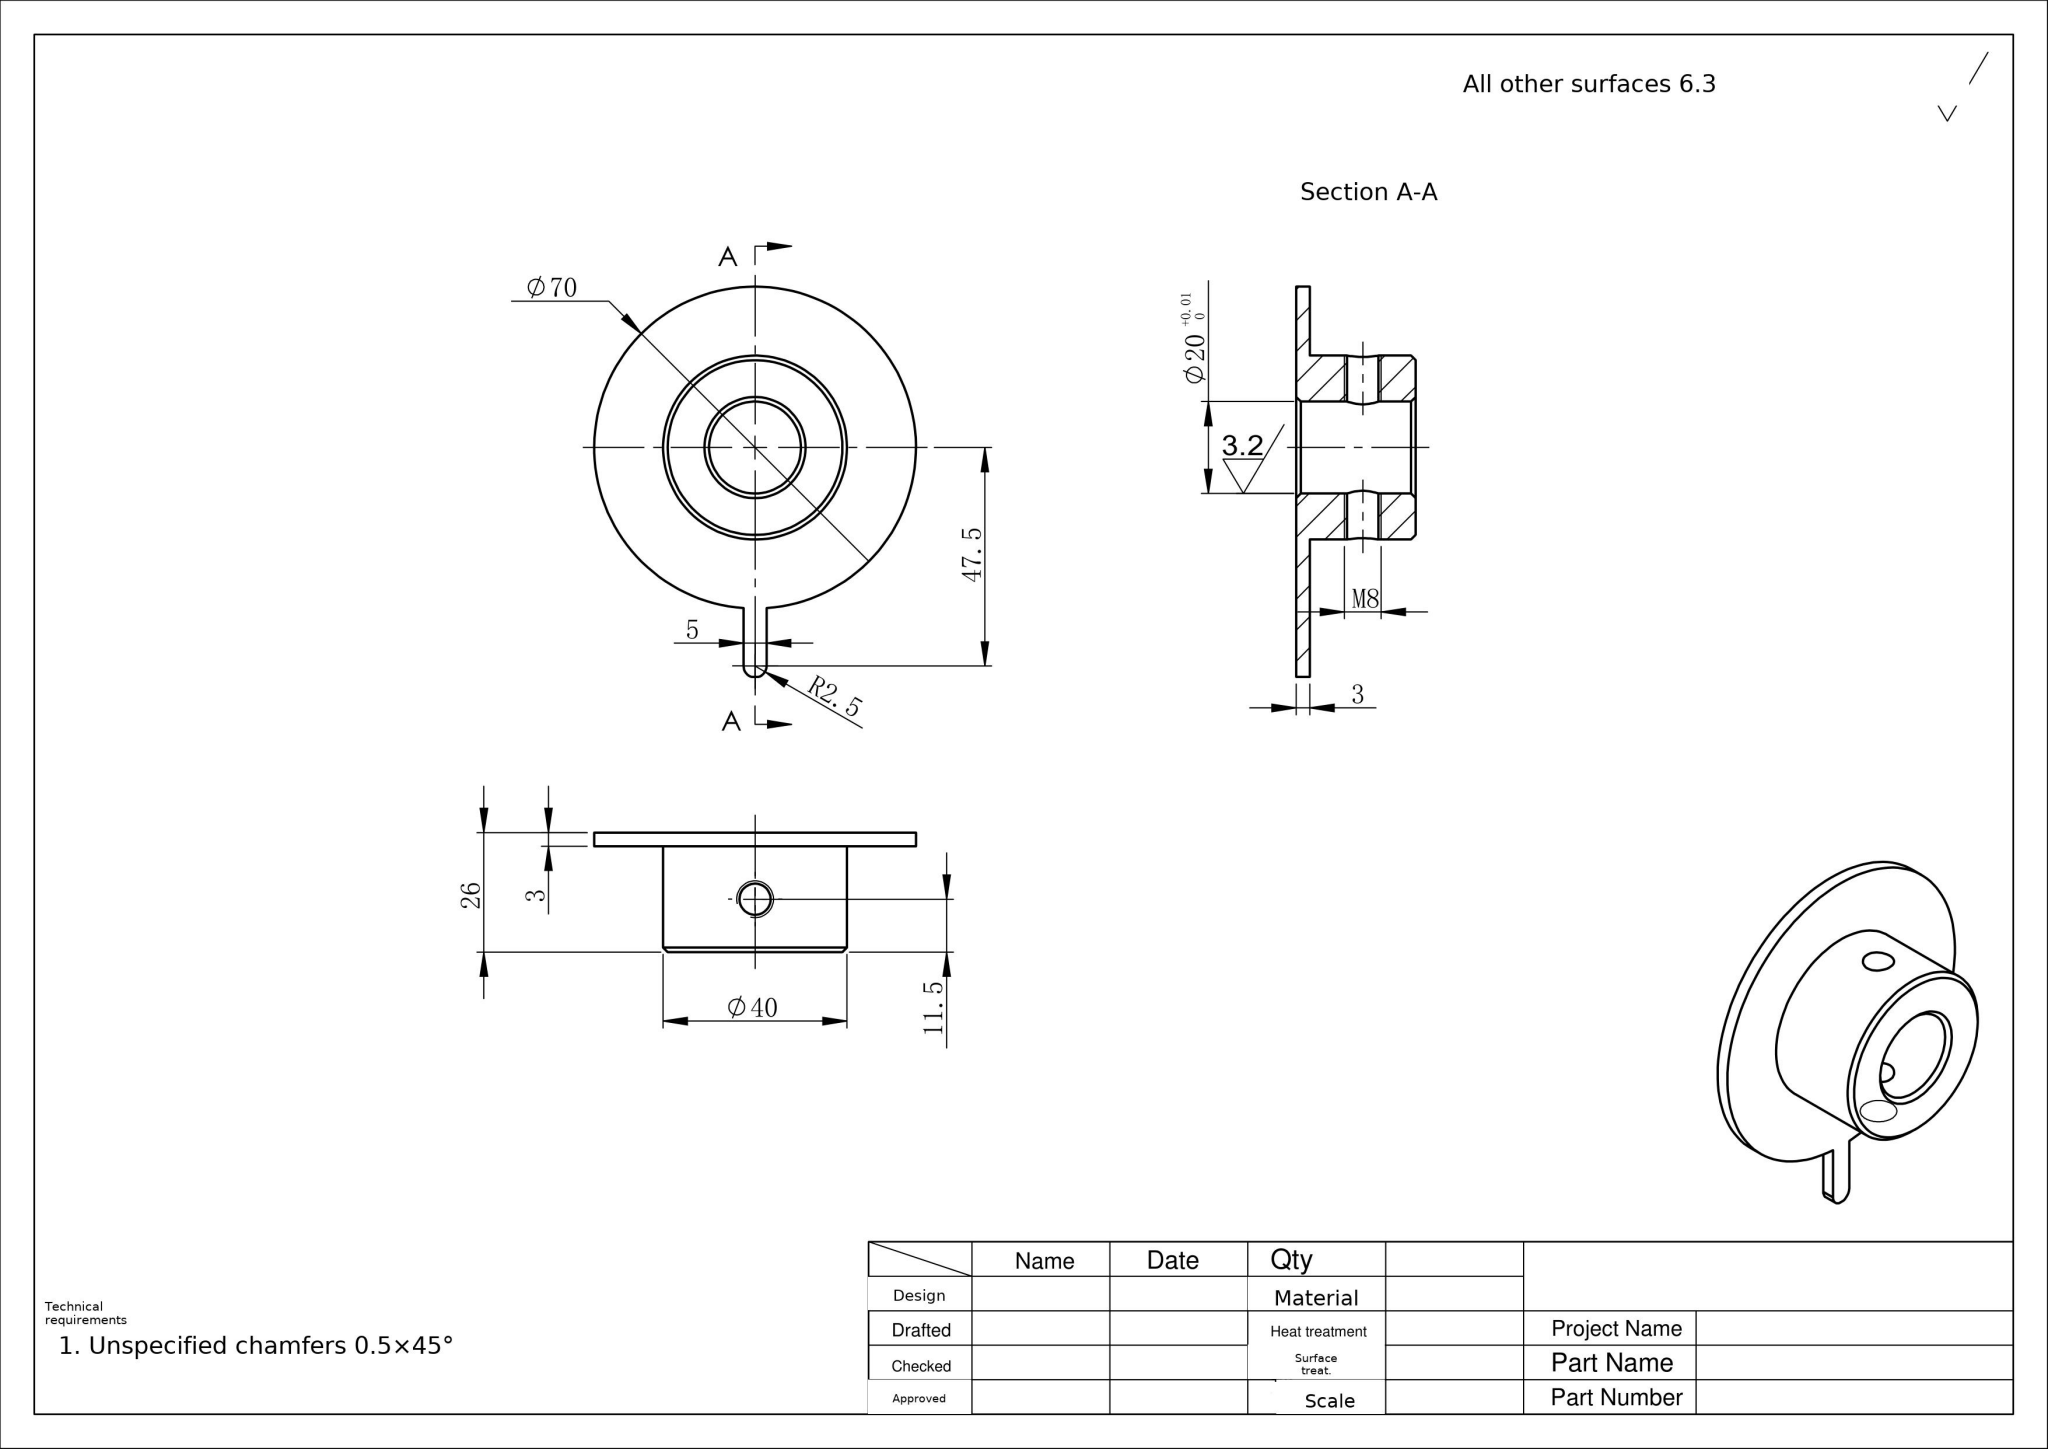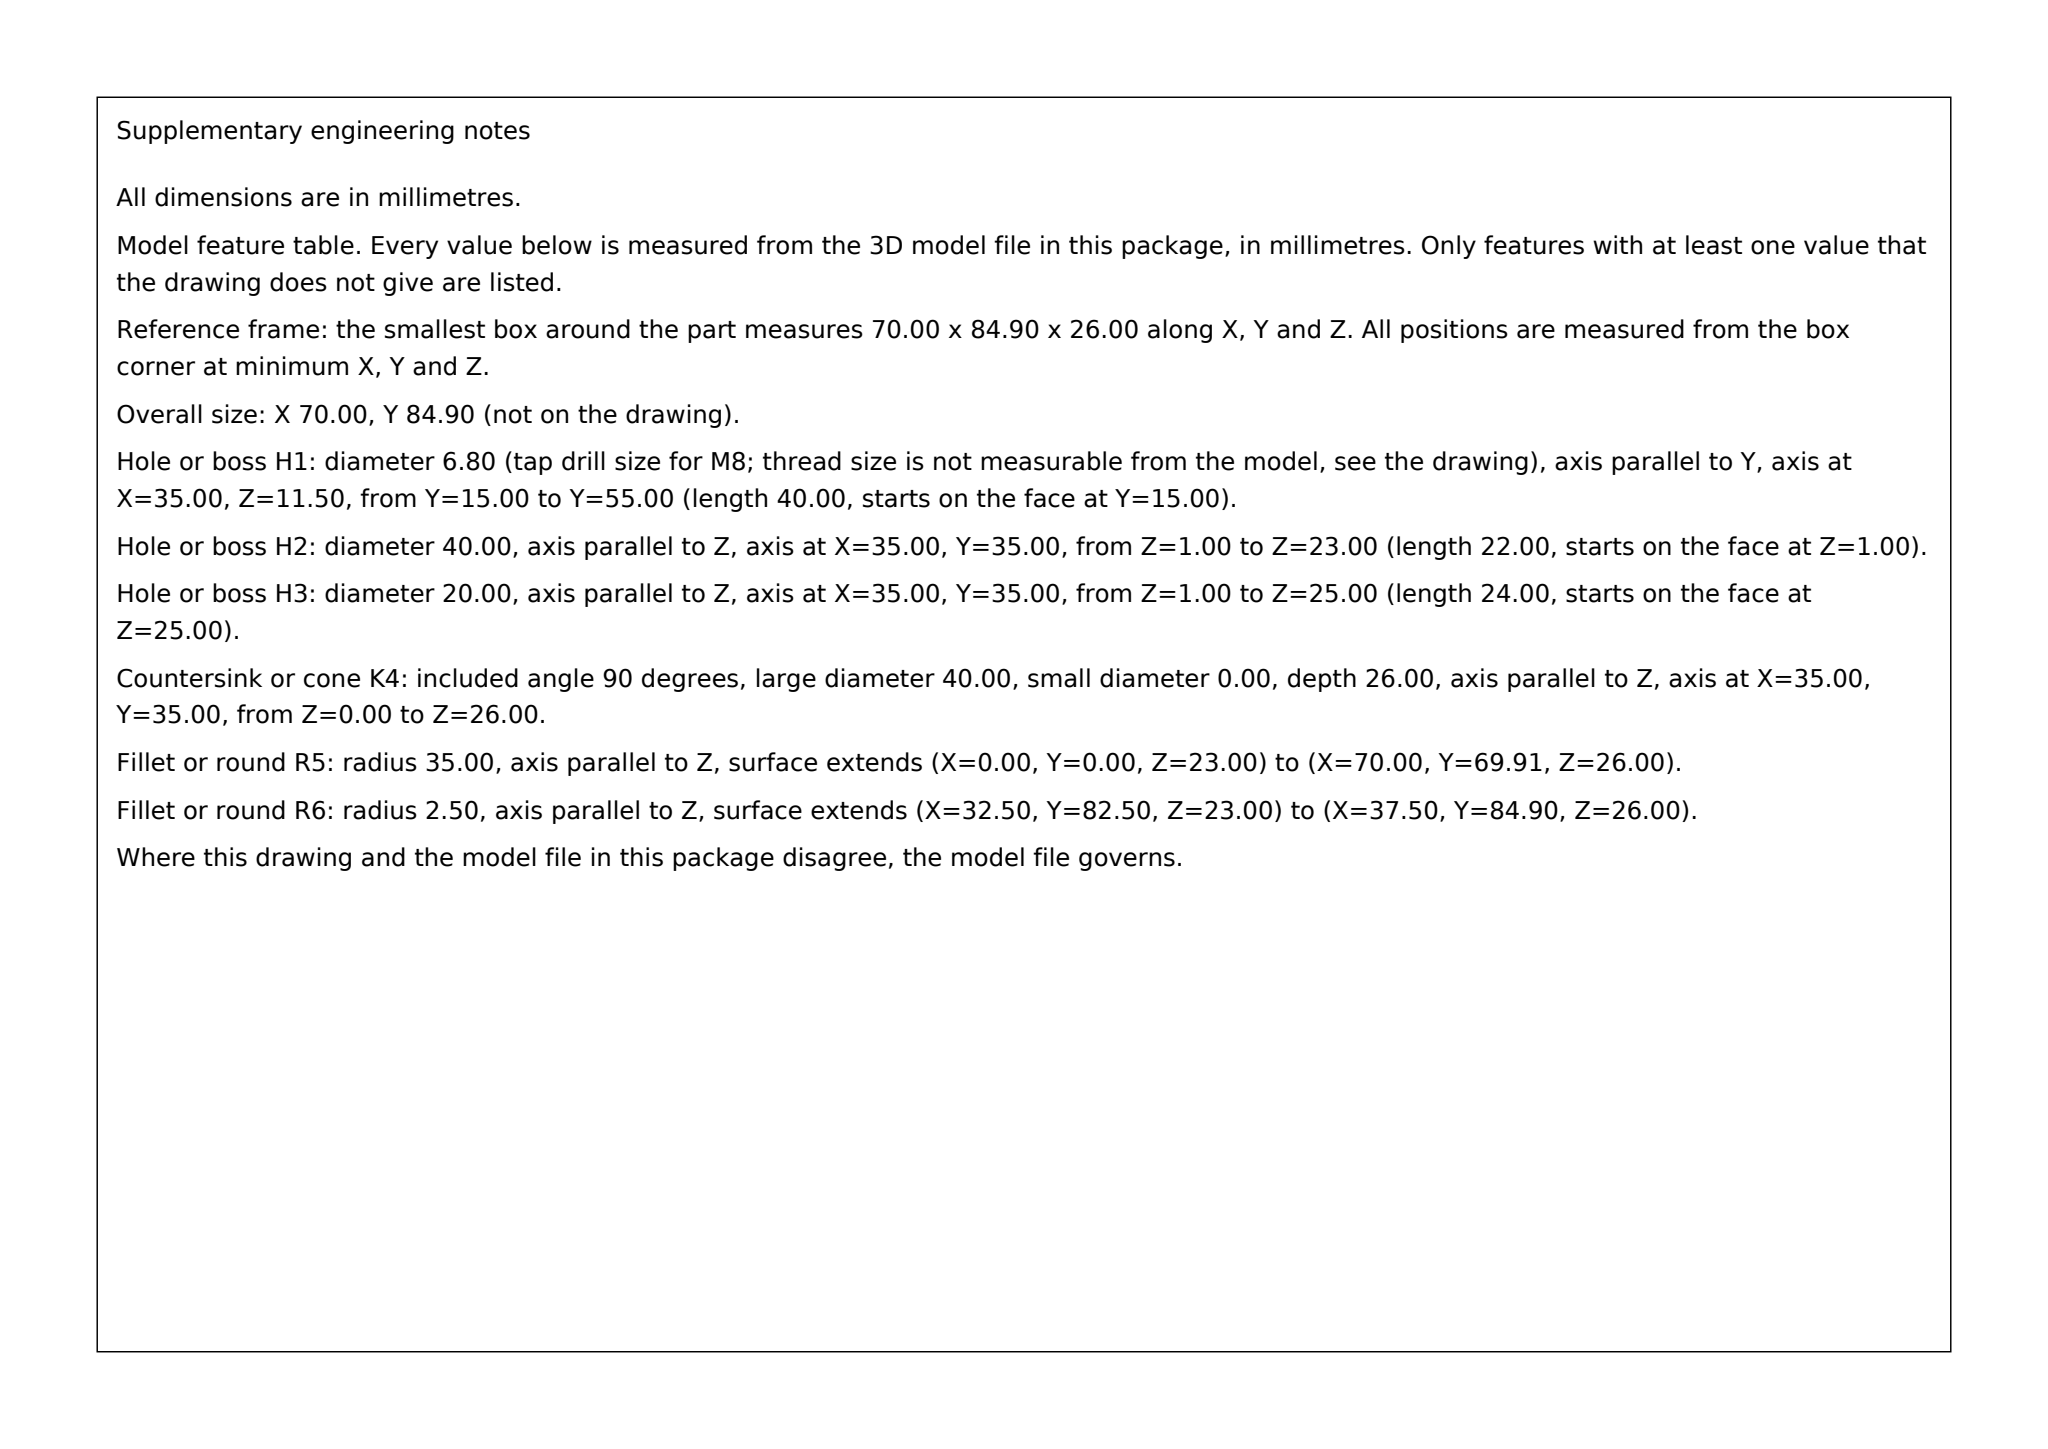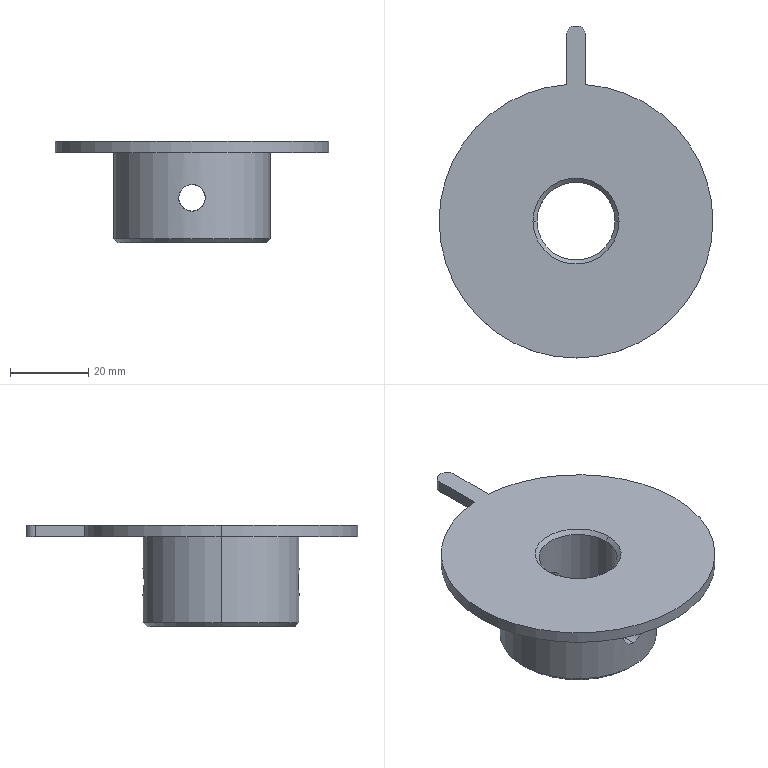Part | SolidWorks | mm | 1 solid | 25 faces | box 70 x 84.9 x 26 mm | volume 31639 mm3 | cylinder 13 | cone 6 | plane 6 | commonest cylinder face diameters 6.8 x4 70 x3 20 x2 40 x2 5 x2